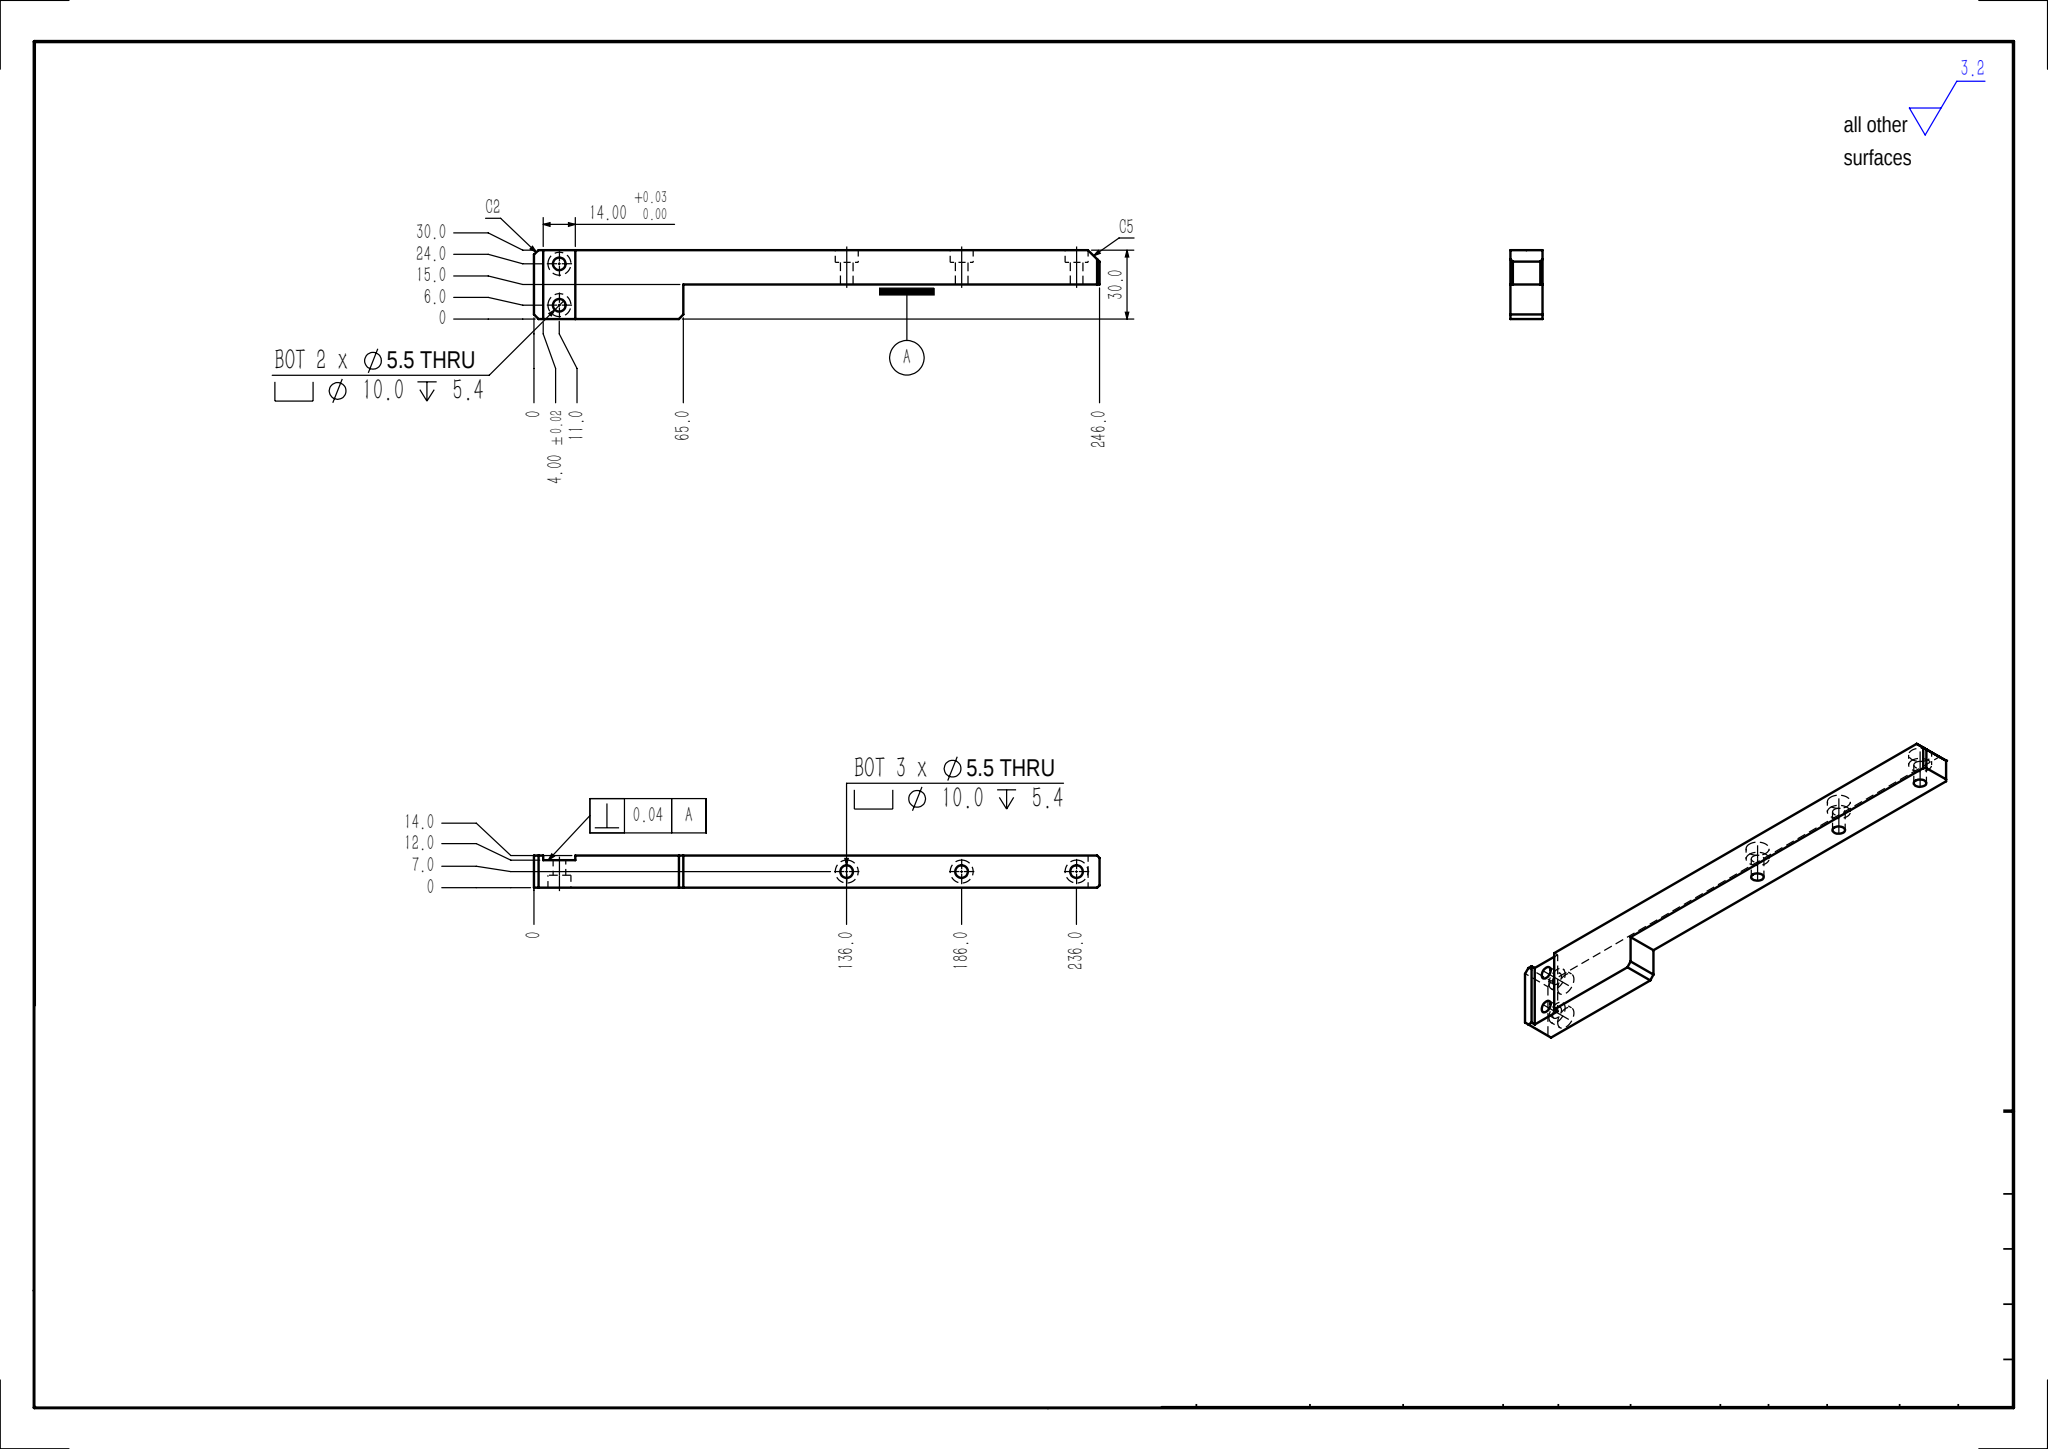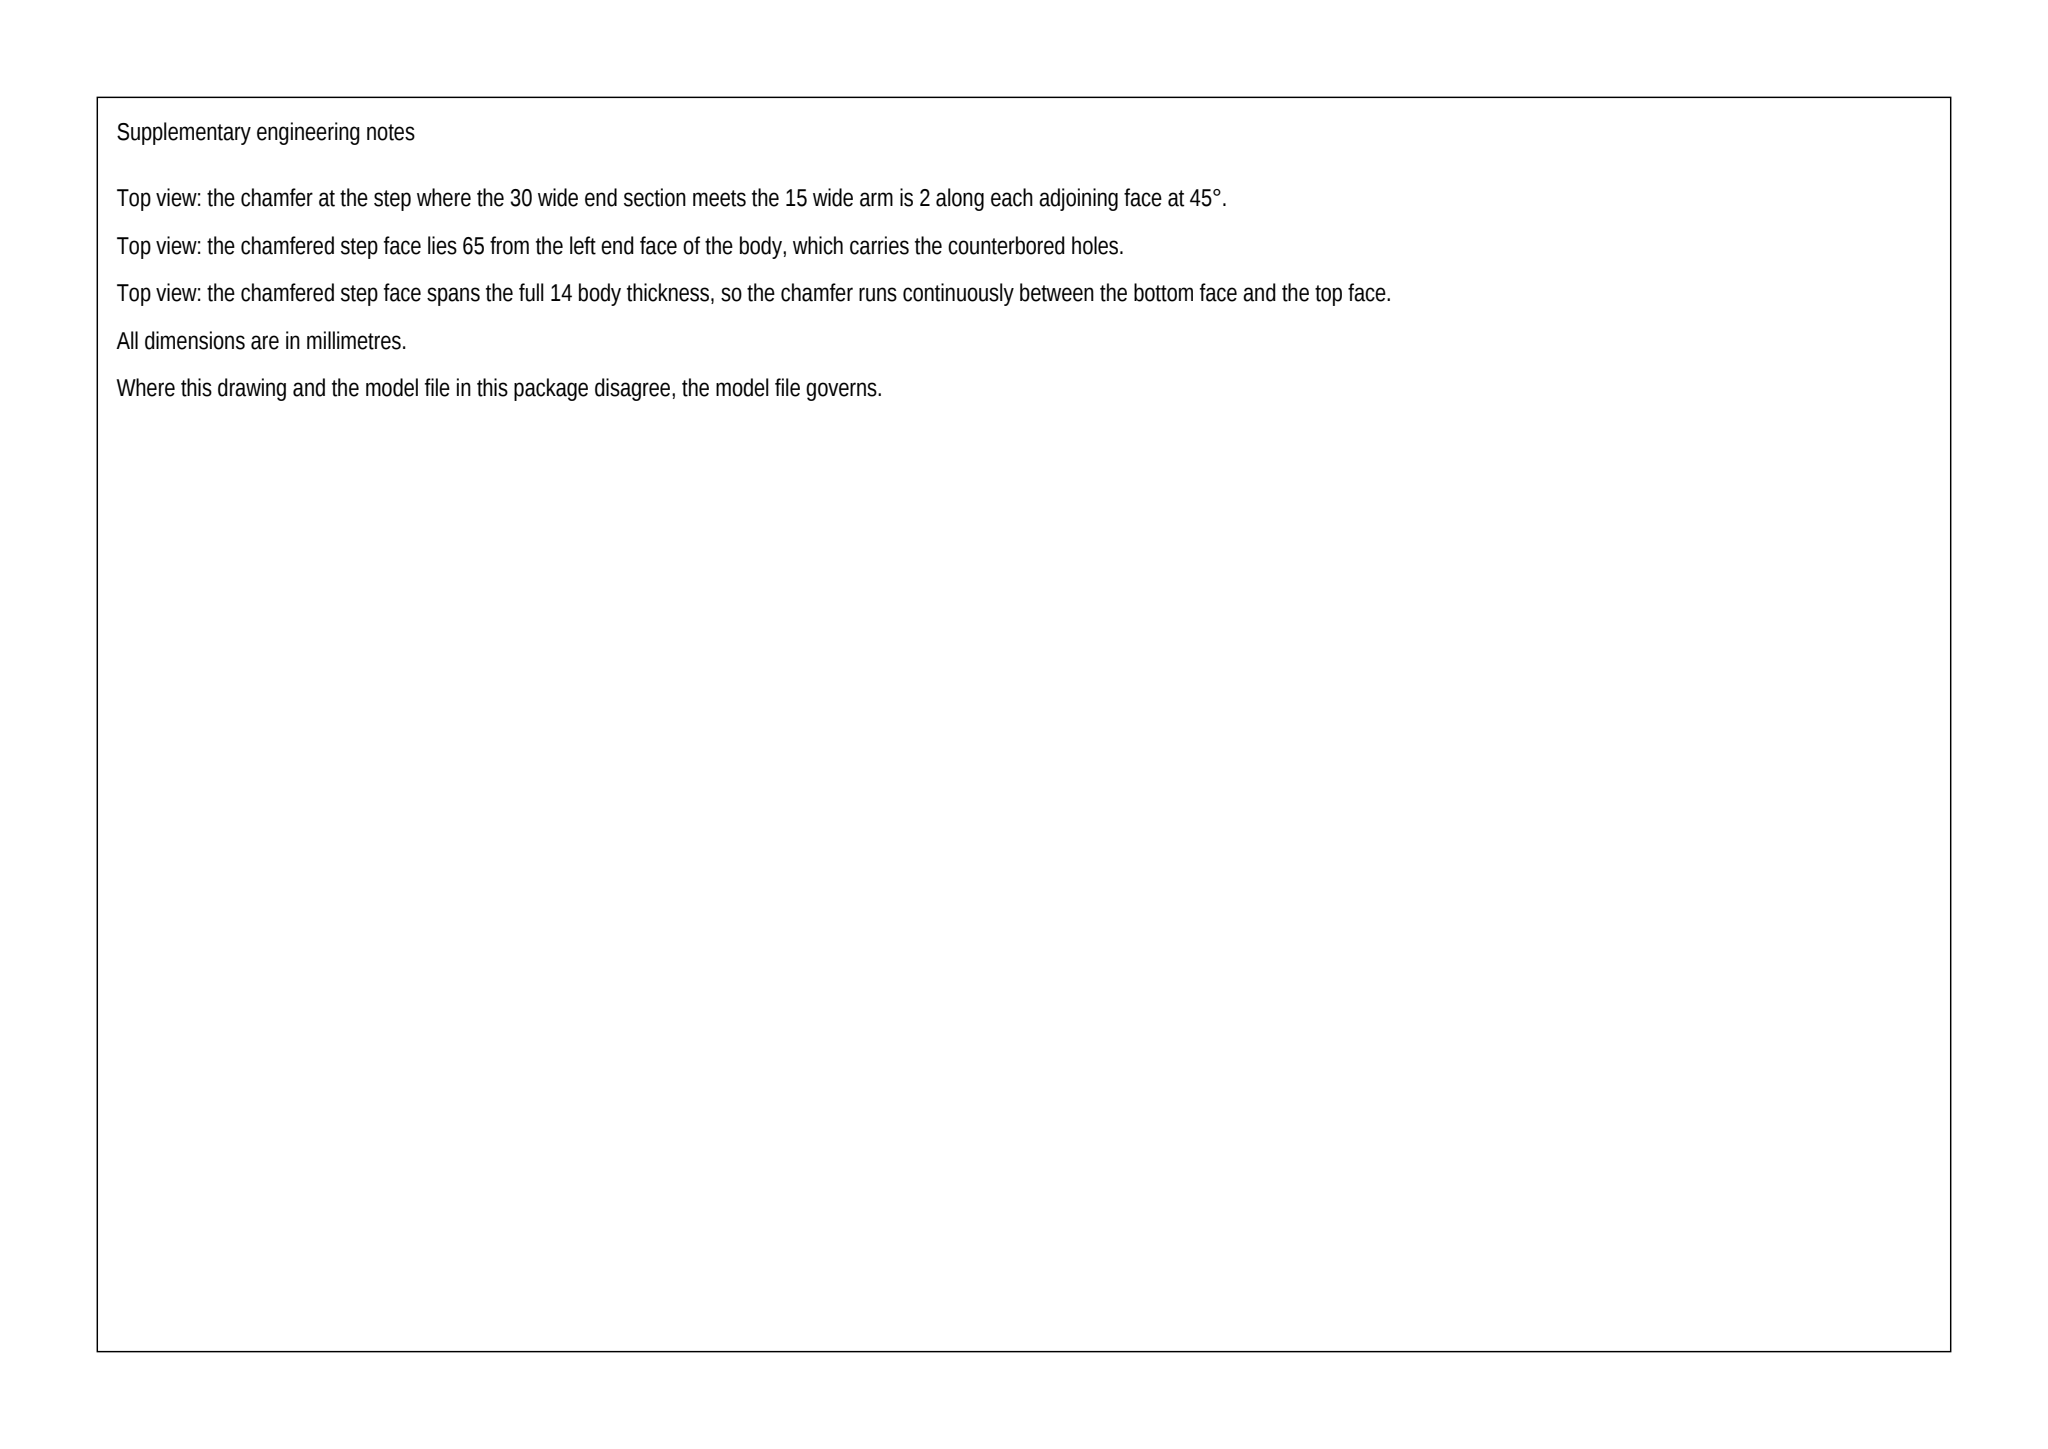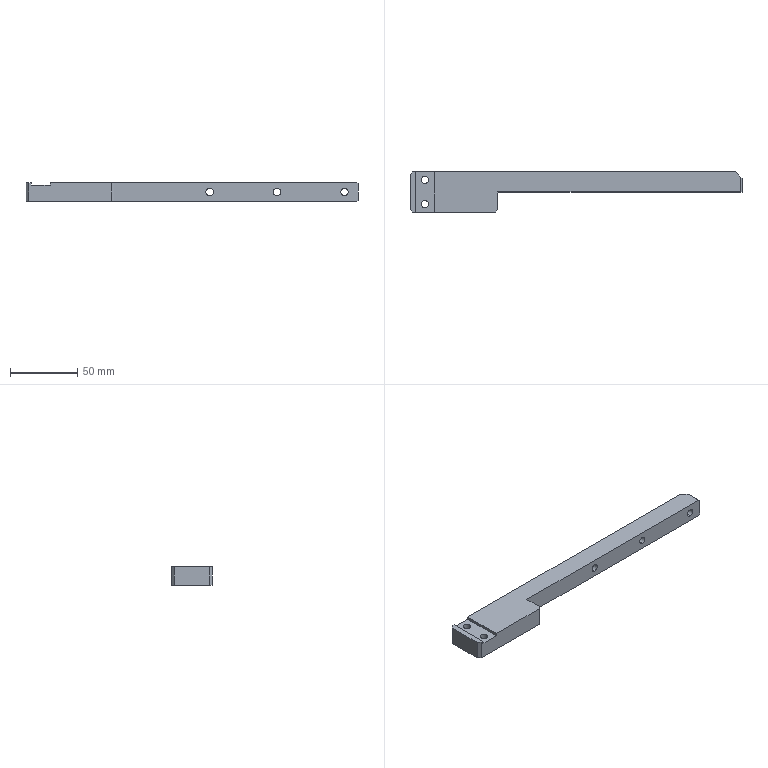Part | SolidWorks | mm | 1 solid | 43 faces | box 246 x 30 x 14 mm | volume 61082 mm3 | plane 23 | cylinder 20 | commonest cylinder face diameters 10 x10 5.5 x10